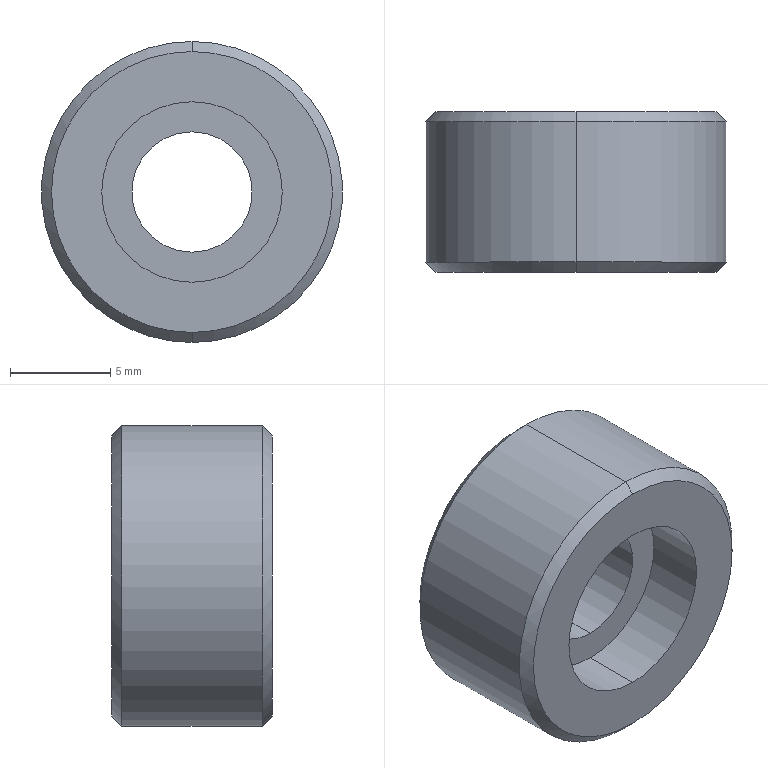Component | SolidWorks | J-TRD899MINI-2213-06SpringAdjustmentWasher-3 | 1 solid | 13 faces | box 15 x 8 x 15 mm | volume 1070 mm3 | cylinder 6 | cone 4 | plane 3 | commonest cylinder face diameters 6 x2 9 x2 15 x2 | material 45
build123d program:
from build123d import *

# Parameters (mm, degrees)
M6_TAPPED_HOLE1_D = 6
CHAMFER1_SIZE     = 0.5


with BuildPart() as part:
    # Sketch1 → Revolve1 (revolve)
    with BuildSketch(Plane.XY, mode=Mode.PRIVATE) as revolve1_sk:
        Polygon((0, 0), (7.5, 0), (7.5, -8), (4.5, -8), (4.5, -5), (0, -5), align=None)
    revolve(revolve1_sk.sketch.rotate(Axis((0, 0, 0), (0, -1, 0)), 90), axis=Axis((0, 0, 0), (0, -1, 0)))

    # M6 Tapped Hole1 (through all)
    with Locations(Plane(origin=(0, 0, 0), x_dir=(1, 0, 0), z_dir=(0, 1, 0))):
        with Locations((0, 0)):
            Hole(M6_TAPPED_HOLE1_D / 2)

    # Chamfer1
    chamfer1_edges = [part.edges().sort_by_distance(p)[0] for p in [
        (0, -8, -7.5),
        (0, 0, -7.5),
    ]]
    chamfer(chamfer1_edges, length=CHAMFER1_SIZE)


solid = part.part

# Placed as in the assembly
solid = solid.moved(Location((-121.663, 49.996, 191.5), (0, 0, 0)))
STEP:
#1=COLOUR_RGB('',0.7922,0.8196,0.9333);
#2=FILL_AREA_STYLE_COLOUR('',#1);
#3=FILL_AREA_STYLE('',(#2));
#4=SURFACE_STYLE_FILL_AREA(#3);
#5=SURFACE_SIDE_STYLE('',(#4));
#6=SURFACE_STYLE_USAGE(.BOTH.,#5);
#7=PRESENTATION_STYLE_ASSIGNMENT((#6));
#8=CARTESIAN_POINT('',(-4.79,1.968,7.815));
#9=VERTEX_POINT('',#8);
#10=CARTESIAN_POINT('',(-4.79,1.968,7.264));
#11=VERTEX_POINT('',#10);
#12=CARTESIAN_POINT('',(-4.79,1.968,7.539));
#13=DIRECTION('',(0.,1.,0.));
#14=DIRECTION('',(0.,0.,-1.));
#15=AXIS2_PLACEMENT_3D('',#12,#13,#14);
#16=CIRCLE('',#15,0.2756);
#17=EDGE_CURVE('',#9,#11,#16,.T.);
#18=ORIENTED_EDGE('',*,*,#17,.F.);
#19=CARTESIAN_POINT('',(-4.79,1.949,7.835));
#20=VERTEX_POINT('',#19);
#21=CARTESIAN_POINT('',(-4.79,1.968,7.815));
#22=DIRECTION('',(0.,-0.7071,0.7071));
#23=VECTOR('',#22,39.37);
#24=LINE('',#21,#23);
#25=EDGE_CURVE('',#9,#20,#24,.T.);
#26=ORIENTED_EDGE('',*,*,#25,.T.);
#27=CARTESIAN_POINT('',(-4.79,1.949,7.244));
#28=VERTEX_POINT('',#27);
#29=CARTESIAN_POINT('',(-4.79,1.949,7.539));
#30=DIRECTION('',(0.,-1.,0.));
#31=DIRECTION('',(0.,0.,-1.));
#32=AXIS2_PLACEMENT_3D('',#29,#30,#31);
#33=CIRCLE('',#32,0.2953);
#34=EDGE_CURVE('',#28,#20,#33,.T.);
#35=ORIENTED_EDGE('',*,*,#34,.F.);
#36=CARTESIAN_POINT('',(-4.79,1.968,7.264));
#37=DIRECTION('',(0.,-0.7071,-0.7071));
#38=VECTOR('',#37,39.37);
#39=LINE('',#36,#38);
#40=EDGE_CURVE('',#11,#28,#39,.T.);
#41=ORIENTED_EDGE('',*,*,#40,.F.);
#42=EDGE_LOOP('',(#18,#26,#35,#41));
#43=FACE_OUTER_BOUND('',#42,.T.);
#44=CARTESIAN_POINT('',(-4.79,1.968,7.539));
#45=DIRECTION('',(0.,-1.,0.));
#46=DIRECTION('',(0.,0.,-1.));
#47=AXIS2_PLACEMENT_3D('',#44,#45,#46);
#48=CONICAL_SURFACE('',#47,0.2756,0.7854);
#49=ADVANCED_FACE('',(#43),#48,.T.);
#50=CARTESIAN_POINT('',(-4.79,1.653,7.264));
#51=VERTEX_POINT('',#50);
#52=CARTESIAN_POINT('',(-4.79,1.653,7.815));
#53=VERTEX_POINT('',#52);
#54=CARTESIAN_POINT('',(-4.79,1.653,7.539));
#55=DIRECTION('',(0.,-1.,0.));
#56=DIRECTION('',(0.,0.,1.));
#57=AXIS2_PLACEMENT_3D('',#54,#55,#56);
#58=CIRCLE('',#57,0.2756);
#59=EDGE_CURVE('',#51,#53,#58,.T.);
#60=ORIENTED_EDGE('',*,*,#59,.F.);
#61=CARTESIAN_POINT('',(-4.79,1.673,7.244));
#62=VERTEX_POINT('',#61);
#63=CARTESIAN_POINT('',(-4.79,1.673,7.244));
#64=DIRECTION('',(0.,0.7071,-0.7071));
#65=VECTOR('',#64,39.37);
#66=LINE('',#63,#65);
#67=EDGE_CURVE('',#51,#62,#66,.T.);
#68=ORIENTED_EDGE('',*,*,#67,.T.);
#69=CARTESIAN_POINT('',(-4.79,1.673,7.835));
#70=VERTEX_POINT('',#69);
#71=CARTESIAN_POINT('',(-4.79,1.673,7.539));
#72=DIRECTION('',(0.,1.,0.));
#73=DIRECTION('',(0.,0.,1.));
#74=AXIS2_PLACEMENT_3D('',#71,#72,#73);
#75=CIRCLE('',#74,0.2953);
#76=EDGE_CURVE('',#70,#62,#75,.T.);
#77=ORIENTED_EDGE('',*,*,#76,.F.);
#78=CARTESIAN_POINT('',(-4.79,1.673,7.835));
#79=DIRECTION('',(0.,0.7071,0.7071));
#80=VECTOR('',#79,39.37);
#81=LINE('',#78,#80);
#82=EDGE_CURVE('',#53,#70,#81,.T.);
#83=ORIENTED_EDGE('',*,*,#82,.F.);
#84=EDGE_LOOP('',(#60,#68,#77,#83));
#85=FACE_OUTER_BOUND('',#84,.T.);
#86=CARTESIAN_POINT('',(-4.79,1.673,7.539));
#87=DIRECTION('',(0.,1.,0.));
#88=DIRECTION('',(0.,0.,1.));
#89=AXIS2_PLACEMENT_3D('',#86,#87,#88);
#90=CONICAL_SURFACE('',#89,0.2953,0.7854);
#91=ADVANCED_FACE('',(#85),#90,.T.);
#92=CARTESIAN_POINT('',(-4.79,1.771,7.421));
#93=VERTEX_POINT('',#92);
#94=CARTESIAN_POINT('',(-4.79,1.771,7.657));
#95=VERTEX_POINT('',#94);
#96=CARTESIAN_POINT('',(-4.79,1.771,7.539));
#97=DIRECTION('',(0.,1.,0.));
#98=DIRECTION('',(0.,0.,1.));
#99=AXIS2_PLACEMENT_3D('',#96,#97,#98);
#100=CIRCLE('',#99,0.1181);
#101=EDGE_CURVE('',#93,#95,#100,.T.);
#102=ORIENTED_EDGE('',*,*,#101,.F.);
#103=CARTESIAN_POINT('',(-4.79,1.968,7.421));
#104=VERTEX_POINT('',#103);
#105=CARTESIAN_POINT('',(-4.79,1.968,7.421));
#106=DIRECTION('',(0.,1.,0.));
#107=VECTOR('',#106,39.37);
#108=LINE('',#105,#107);
#109=EDGE_CURVE('',#93,#104,#108,.T.);
#110=ORIENTED_EDGE('',*,*,#109,.T.);
#111=CARTESIAN_POINT('',(-4.79,1.968,7.657));
#112=VERTEX_POINT('',#111);
#113=CARTESIAN_POINT('',(-4.79,1.968,7.539));
#114=DIRECTION('',(0.,1.,0.));
#115=DIRECTION('',(0.,0.,1.));
#116=AXIS2_PLACEMENT_3D('',#113,#114,#115);
#117=CIRCLE('',#116,0.1181);
#118=EDGE_CURVE('',#104,#112,#117,.T.);
#119=ORIENTED_EDGE('',*,*,#118,.T.);
#120=CARTESIAN_POINT('',(-4.79,1.968,7.657));
#121=DIRECTION('',(0.,1.,0.));
#122=VECTOR('',#121,39.37);
#123=LINE('',#120,#122);
#124=EDGE_CURVE('',#95,#112,#123,.T.);
#125=ORIENTED_EDGE('',*,*,#124,.F.);
#126=EDGE_LOOP('',(#102,#110,#119,#125));
#127=FACE_OUTER_BOUND('',#126,.T.);
#128=CARTESIAN_POINT('',(-4.79,1.968,7.539));
#129=DIRECTION('',(0.,1.,0.));
#130=DIRECTION('',(0.,0.,1.));
#131=AXIS2_PLACEMENT_3D('',#128,#129,#130);
#132=CYLINDRICAL_SURFACE('',#131,0.1181);
#133=ADVANCED_FACE('',(#127),#132,.F.);
#134=CARTESIAN_POINT('',(-4.79,1.653,7.362));
#135=VERTEX_POINT('',#134);
#136=CARTESIAN_POINT('',(-4.79,1.653,7.717));
#137=VERTEX_POINT('',#136);
#138=CARTESIAN_POINT('',(-4.79,1.653,7.539));
#139=DIRECTION('',(0.,1.,0.));
#140=DIRECTION('',(0.,0.,1.));
#141=AXIS2_PLACEMENT_3D('',#138,#139,#140);
#142=CIRCLE('',#141,0.1772);
#143=EDGE_CURVE('',#135,#137,#142,.T.);
#144=ORIENTED_EDGE('',*,*,#143,.F.);
#145=CARTESIAN_POINT('',(-4.79,1.771,7.362));
#146=VERTEX_POINT('',#145);
#147=CARTESIAN_POINT('',(-4.79,1.968,7.362));
#148=DIRECTION('',(0.,1.,0.));
#149=VECTOR('',#148,39.37);
#150=LINE('',#147,#149);
#151=EDGE_CURVE('',#135,#146,#150,.T.);
#152=ORIENTED_EDGE('',*,*,#151,.T.);
#153=CARTESIAN_POINT('',(-4.79,1.771,7.717));
#154=VERTEX_POINT('',#153);
#155=CARTESIAN_POINT('',(-4.79,1.771,7.539));
#156=DIRECTION('',(0.,1.,0.));
#157=DIRECTION('',(0.,0.,1.));
#158=AXIS2_PLACEMENT_3D('',#155,#156,#157);
#159=CIRCLE('',#158,0.1772);
#160=EDGE_CURVE('',#146,#154,#159,.T.);
#161=ORIENTED_EDGE('',*,*,#160,.T.);
#162=CARTESIAN_POINT('',(-4.79,1.968,7.717));
#163=DIRECTION('',(0.,1.,0.));
#164=VECTOR('',#163,39.37);
#165=LINE('',#162,#164);
#166=EDGE_CURVE('',#137,#154,#165,.T.);
#167=ORIENTED_EDGE('',*,*,#166,.F.);
#168=EDGE_LOOP('',(#144,#152,#161,#167));
#169=FACE_OUTER_BOUND('',#168,.T.);
#170=CARTESIAN_POINT('',(-4.79,1.968,7.539));
#171=DIRECTION('',(0.,1.,0.));
#172=DIRECTION('',(0.,0.,1.));
#173=AXIS2_PLACEMENT_3D('',#170,#171,#172);
#174=CYLINDRICAL_SURFACE('',#173,0.1772);
#175=ADVANCED_FACE('',(#169),#174,.F.);
#176=ORIENTED_EDGE('',*,*,#76,.T.);
#177=CARTESIAN_POINT('',(-4.79,1.968,7.244));
#178=DIRECTION('',(0.,1.,0.));
#179=VECTOR('',#178,39.37);
#180=LINE('',#177,#179);
#181=EDGE_CURVE('',#62,#28,#180,.T.);
#182=ORIENTED_EDGE('',*,*,#181,.T.);
#183=ORIENTED_EDGE('',*,*,#34,.T.);
#184=CARTESIAN_POINT('',(-4.79,1.968,7.835));
#185=DIRECTION('',(0.,1.,0.));
#186=VECTOR('',#185,39.37);
#187=LINE('',#184,#186);
#188=EDGE_CURVE('',#70,#20,#187,.T.);
#189=ORIENTED_EDGE('',*,*,#188,.F.);
#190=EDGE_LOOP('',(#176,#182,#183,#189));
#191=FACE_OUTER_BOUND('',#190,.T.);
#192=CARTESIAN_POINT('',(-4.79,1.968,7.539));
#193=DIRECTION('',(0.,1.,0.));
#194=DIRECTION('',(0.,0.,1.));
#195=AXIS2_PLACEMENT_3D('',#192,#193,#194);
#196=CYLINDRICAL_SURFACE('',#195,0.2953);
#197=ADVANCED_FACE('',(#191),#196,.T.);
#198=CARTESIAN_POINT('',(-4.79,1.968,7.539));
#199=DIRECTION('',(0.,1.,0.));
#200=DIRECTION('',(0.,0.,-1.));
#201=AXIS2_PLACEMENT_3D('',#198,#199,#200);
#202=CIRCLE('',#201,0.2756);
#203=EDGE_CURVE('',#11,#9,#202,.T.);
#204=ORIENTED_EDGE('',*,*,#203,.T.);
#205=ORIENTED_EDGE('',*,*,#17,.T.);
#206=EDGE_LOOP('',(#204,#205));
#207=FACE_OUTER_BOUND('',#206,.T.);
#208=CARTESIAN_POINT('',(-4.79,1.968,7.539));
#209=DIRECTION('',(0.,1.,0.));
#210=DIRECTION('',(0.,0.,1.));
#211=AXIS2_PLACEMENT_3D('',#208,#209,#210);
#212=CIRCLE('',#211,0.1181);
#213=EDGE_CURVE('',#112,#104,#212,.T.);
#214=ORIENTED_EDGE('',*,*,#213,.F.);
#215=ORIENTED_EDGE('',*,*,#118,.F.);
#216=EDGE_LOOP('',(#214,#215));
#217=FACE_BOUND('',#216,.T.);
#218=CARTESIAN_POINT('',(-4.79,1.968,7.539));
#219=DIRECTION('',(0.,-1.,0.));
#220=DIRECTION('',(0.,0.,-1.));
#221=AXIS2_PLACEMENT_3D('',#218,#219,#220);
#222=PLANE('',#221);
#223=ADVANCED_FACE('',(#207,#217),#222,.F.);
#224=ORIENTED_EDGE('',*,*,#181,.F.);
#225=CARTESIAN_POINT('',(-4.79,1.673,7.539));
#226=DIRECTION('',(0.,1.,0.));
#227=DIRECTION('',(0.,0.,1.));
#228=AXIS2_PLACEMENT_3D('',#225,#226,#227);
#229=CIRCLE('',#228,0.2953);
#230=EDGE_CURVE('',#62,#70,#229,.T.);
#231=ORIENTED_EDGE('',*,*,#230,.T.);
#232=ORIENTED_EDGE('',*,*,#188,.T.);
#233=CARTESIAN_POINT('',(-4.79,1.949,7.539));
#234=DIRECTION('',(0.,-1.,0.));
#235=DIRECTION('',(0.,0.,-1.));
#236=AXIS2_PLACEMENT_3D('',#233,#234,#235);
#237=CIRCLE('',#236,0.2953);
#238=EDGE_CURVE('',#20,#28,#237,.T.);
#239=ORIENTED_EDGE('',*,*,#238,.T.);
#240=EDGE_LOOP('',(#224,#231,#232,#239));
#241=FACE_OUTER_BOUND('',#240,.T.);
#242=CARTESIAN_POINT('',(-4.79,1.968,7.539));
#243=DIRECTION('',(0.,1.,0.));
#244=DIRECTION('',(0.,0.,1.));
#245=AXIS2_PLACEMENT_3D('',#242,#243,#244);
#246=CYLINDRICAL_SURFACE('',#245,0.2953);
#247=ADVANCED_FACE('',(#241),#246,.T.);
#248=CARTESIAN_POINT('',(-4.79,1.653,7.539));
#249=DIRECTION('',(0.,-1.,0.));
#250=DIRECTION('',(0.,0.,1.));
#251=AXIS2_PLACEMENT_3D('',#248,#249,#250);
#252=CIRCLE('',#251,0.2756);
#253=EDGE_CURVE('',#53,#51,#252,.T.);
#254=ORIENTED_EDGE('',*,*,#253,.T.);
#255=ORIENTED_EDGE('',*,*,#59,.T.);
#256=EDGE_LOOP('',(#254,#255));
#257=FACE_OUTER_BOUND('',#256,.T.);
#258=CARTESIAN_POINT('',(-4.79,1.653,7.539));
#259=DIRECTION('',(0.,1.,0.));
#260=DIRECTION('',(0.,0.,1.));
#261=AXIS2_PLACEMENT_3D('',#258,#259,#260);
#262=CIRCLE('',#261,0.1772);
#263=EDGE_CURVE('',#137,#135,#262,.T.);
#264=ORIENTED_EDGE('',*,*,#263,.T.);
#265=ORIENTED_EDGE('',*,*,#143,.T.);
#266=EDGE_LOOP('',(#264,#265));
#267=FACE_BOUND('',#266,.T.);
#268=CARTESIAN_POINT('',(-4.495,1.653,7.539));
#269=DIRECTION('',(0.,1.,0.));
#270=DIRECTION('',(0.,0.,1.));
#271=AXIS2_PLACEMENT_3D('',#268,#269,#270);
#272=PLANE('',#271);
#273=ADVANCED_FACE('',(#257,#267),#272,.F.);
#274=ORIENTED_EDGE('',*,*,#151,.F.);
#275=ORIENTED_EDGE('',*,*,#263,.F.);
#276=ORIENTED_EDGE('',*,*,#166,.T.);
#277=CARTESIAN_POINT('',(-4.79,1.771,7.539));
#278=DIRECTION('',(0.,1.,0.));
#279=DIRECTION('',(0.,0.,1.));
#280=AXIS2_PLACEMENT_3D('',#277,#278,#279);
#281=CIRCLE('',#280,0.1772);
#282=EDGE_CURVE('',#154,#146,#281,.T.);
#283=ORIENTED_EDGE('',*,*,#282,.T.);
#284=EDGE_LOOP('',(#274,#275,#276,#283));
#285=FACE_OUTER_BOUND('',#284,.T.);
#286=CARTESIAN_POINT('',(-4.79,1.968,7.539));
#287=DIRECTION('',(0.,1.,0.));
#288=DIRECTION('',(0.,0.,1.));
#289=AXIS2_PLACEMENT_3D('',#286,#287,#288);
#290=CYLINDRICAL_SURFACE('',#289,0.1772);
#291=ADVANCED_FACE('',(#285),#290,.F.);
#292=CARTESIAN_POINT('',(-4.79,1.771,7.539));
#293=DIRECTION('',(0.,1.,0.));
#294=DIRECTION('',(0.,0.,1.));
#295=AXIS2_PLACEMENT_3D('',#292,#293,#294);
#296=CIRCLE('',#295,0.1181);
#297=EDGE_CURVE('',#95,#93,#296,.T.);
#298=ORIENTED_EDGE('',*,*,#297,.T.);
#299=ORIENTED_EDGE('',*,*,#101,.T.);
#300=EDGE_LOOP('',(#298,#299));
#301=FACE_BOUND('',#300,.T.);
#302=ORIENTED_EDGE('',*,*,#282,.F.);
#303=ORIENTED_EDGE('',*,*,#160,.F.);
#304=EDGE_LOOP('',(#302,#303));
#305=FACE_OUTER_BOUND('',#304,.T.);
#306=CARTESIAN_POINT('',(-4.613,1.771,7.539));
#307=DIRECTION('',(0.,1.,0.));
#308=DIRECTION('',(0.,0.,1.));
#309=AXIS2_PLACEMENT_3D('',#306,#307,#308);
#310=PLANE('',#309);
#311=ADVANCED_FACE('',(#301,#305),#310,.F.);
#312=ORIENTED_EDGE('',*,*,#109,.F.);
#313=ORIENTED_EDGE('',*,*,#297,.F.);
#314=ORIENTED_EDGE('',*,*,#124,.T.);
#315=ORIENTED_EDGE('',*,*,#213,.T.);
#316=EDGE_LOOP('',(#312,#313,#314,#315));
#317=FACE_OUTER_BOUND('',#316,.T.);
#318=CARTESIAN_POINT('',(-4.79,1.968,7.539));
#319=DIRECTION('',(0.,1.,0.));
#320=DIRECTION('',(0.,0.,1.));
#321=AXIS2_PLACEMENT_3D('',#318,#319,#320);
#322=CYLINDRICAL_SURFACE('',#321,0.1181);
#323=ADVANCED_FACE('',(#317),#322,.F.);
#324=ORIENTED_EDGE('',*,*,#67,.F.);
#325=ORIENTED_EDGE('',*,*,#253,.F.);
#326=ORIENTED_EDGE('',*,*,#82,.T.);
#327=ORIENTED_EDGE('',*,*,#230,.F.);
#328=EDGE_LOOP('',(#324,#325,#326,#327));
#329=FACE_OUTER_BOUND('',#328,.T.);
#330=CARTESIAN_POINT('',(-4.79,1.673,7.539));
#331=DIRECTION('',(0.,1.,0.));
#332=DIRECTION('',(0.,0.,1.));
#333=AXIS2_PLACEMENT_3D('',#330,#331,#332);
#334=CONICAL_SURFACE('',#333,0.2953,0.7854);
#335=ADVANCED_FACE('',(#329),#334,.T.);
#336=ORIENTED_EDGE('',*,*,#25,.F.);
#337=ORIENTED_EDGE('',*,*,#203,.F.);
#338=ORIENTED_EDGE('',*,*,#40,.T.);
#339=ORIENTED_EDGE('',*,*,#238,.F.);
#340=EDGE_LOOP('',(#336,#337,#338,#339));
#341=FACE_OUTER_BOUND('',#340,.T.);
#342=CARTESIAN_POINT('',(-4.79,1.968,7.539));
#343=DIRECTION('',(0.,-1.,0.));
#344=DIRECTION('',(0.,0.,-1.));
#345=AXIS2_PLACEMENT_3D('',#342,#343,#344);
#346=CONICAL_SURFACE('',#345,0.2756,0.7854);
#347=ADVANCED_FACE('',(#341),#346,.T.);
#348=CLOSED_SHELL('',(#49,#91,#133,#175,#197,#223,#247,#273,#291,#311,#323,#335,#347));
#349=MANIFOLD_SOLID_BREP('',#348);
#350=STYLED_ITEM('',(#7),#349);
#351=PRESENTATION_LAYER_ASSIGNMENT('','',(#350));
#352=(LENGTH_UNIT()NAMED_UNIT(*)SI_UNIT($,.METRE.));
#353=LENGTH_MEASURE_WITH_UNIT(LENGTH_MEASURE(0.0254),#352);
#354=DIMENSIONAL_EXPONENTS(1.,0.,0.,0.,0.,0.,0.);
#355=(CONVERSION_BASED_UNIT('',#353)LENGTH_UNIT()NAMED_UNIT(#354));
#356=UNCERTAINTY_MEASURE_WITH_UNIT(LENGTH_MEASURE(0.00001),#355,'','');
#357=(NAMED_UNIT(*)PLANE_ANGLE_UNIT()SI_UNIT($,.RADIAN.));
#358=(NAMED_UNIT(*)SI_UNIT($,.STERADIAN.)SOLID_ANGLE_UNIT());
#359=(GEOMETRIC_REPRESENTATION_CONTEXT(3)GLOBAL_UNCERTAINTY_ASSIGNED_CONTEXT((#356))GLOBAL_UNIT_ASSIGNED_CONTEXT((#355,#357,#358))REPRESENTATION_CONTEXT('',''));
#360=MECHANICAL_DESIGN_GEOMETRIC_PRESENTATION_REPRESENTATION('',(#350),#359);
#361=CARTESIAN_POINT('',(0.,0.,0.));
#362=DIRECTION('',(0.,0.,1.));
#363=DIRECTION('',(1.,0.,0.));
#364=AXIS2_PLACEMENT_3D('',#361,#362,#363);
#365=(LENGTH_UNIT()NAMED_UNIT(*)SI_UNIT($,.METRE.));
#366=LENGTH_MEASURE_WITH_UNIT(LENGTH_MEASURE(0.0254),#365);
#367=DIMENSIONAL_EXPONENTS(1.,0.,0.,0.,0.,0.,0.);
#368=(CONVERSION_BASED_UNIT('',#366)LENGTH_UNIT()NAMED_UNIT(#367));
#369=UNCERTAINTY_MEASURE_WITH_UNIT(LENGTH_MEASURE(0.00001),#368,'','');
#370=(NAMED_UNIT(*)PLANE_ANGLE_UNIT()SI_UNIT($,.RADIAN.));
#371=(NAMED_UNIT(*)SI_UNIT($,.STERADIAN.)SOLID_ANGLE_UNIT());
#372=(GEOMETRIC_REPRESENTATION_CONTEXT(3)GLOBAL_UNCERTAINTY_ASSIGNED_CONTEXT((#369))GLOBAL_UNIT_ASSIGNED_CONTEXT((#368,#370,#371))REPRESENTATION_CONTEXT('',''));
#373=ADVANCED_BREP_SHAPE_REPRESENTATION('',(#349,#364),#372);